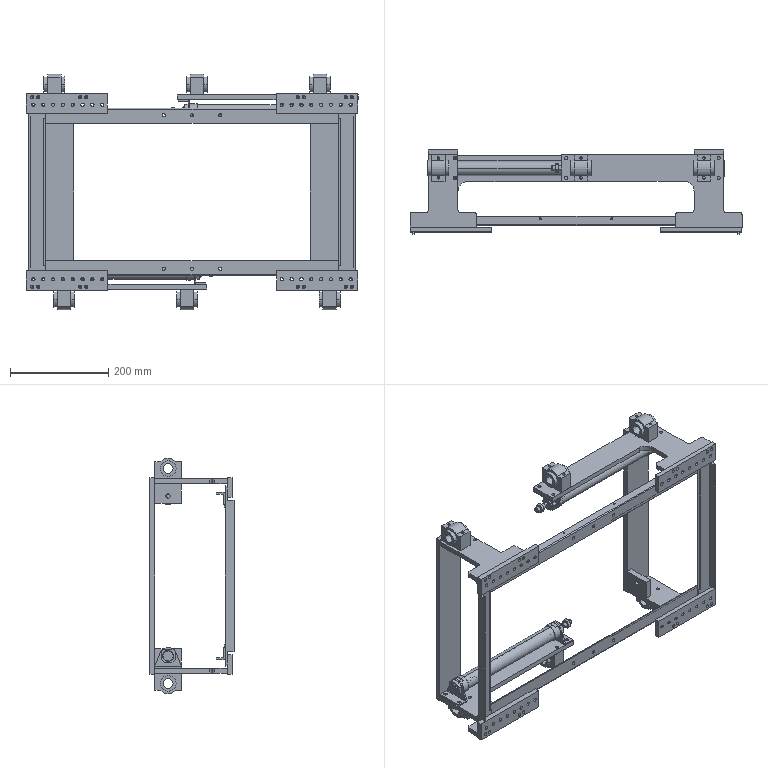Assembly | SolidWorks | mm | 30 component files | 36 solids | 1020 faces | box 675 x 171 x 479 mm | volume 2445017 mm3 | cylinder 492 | plane 356 | cone 140 | torus 32 | commonest cylinder face diameters 6.6 x192 5 x80 32 x32 10 x28 5.2 x24 22 x16 3.3 x16 34 x12
Bill of materials:
AluminumAlloyMiniCylinder-MAL-25x210-S-CM-AIRTAC | 2 | Q235A | Long, slender body of revolution: a plain cylindrical barrel with a wider collar at each end, a short smaller-diameter boss on the rear end, and on the front end a stepped nose with a hex-shaped nut, then a thin protruding rod that carries a second small hex nut and ends in a short stub.
BoxShortLinearBearing-SC20VUU-WERB | 6 |  | Rectangular block with a flat top and a half-round lower side. A cylindrical hub sticks out a short distance from both opposite faces, and a large through-bore runs through the block along the hub axis. Two small holes go down through the top face, one near each end.
CTM-HVS-42-02-27 | 4 | Q235A Cold Rolled Sheet 3mm | L-shaped bent plate bracket. The upright leg tapers to a rounded top and has one large circular hole. The flat base leg is rectangular with two smaller holes. The bend has an inside radius, and the base corners are slightly chamfered.
CTM-HVS-42-02-28 | 2 | Q235A | Thin ring with a large central round bore. The outer profile is a hexagon with its corners cut off by a circle (corner chamfers or rounding), similar in form to a thin jam nut.
CTM-HVS-42-02-29 | 2 | Q235A | Flat plate of uniform thickness with an inverted-L / T-like outline: a long rectangular arm plus a wider foot section at one end. The inside corner is filleted. Four through-holes sit in the face at each end of the long arm, and pairs of holes are drilled into the edge of the foot.
CTM-HVS-42-02-30 | 2 | Q235A | Long, thin rectangular flat plate with five small through-holes near the ends: two at one end plus a third slightly inboard, and two at the opposite end.
CTM-HVS-42-02-31 | 4 | Bakelite | Rectangular flat bar of moderate thickness with a row of eight evenly spaced through-holes along its length. Two extra pairs of holes sit in a second row below.
CTM-HVS-52-OA-02-08-01 | 2 | Q235A | Flat T-shaped plate of uniform thickness. A rectangular stem joins a wider crossbar, with filleted inside corners and rounded outer corners on the crossbar. Four through-holes sit in a rectangular pattern on the stem, and two pairs of holes are drilled into the crossbar's long edge.
CTM-HVS-52-OA-02-14 | 2 | 316L | Long straight member with an L-shaped cross-section: a thin flange plus a perpendicular leg. The leg stops short of both ends, leaving flat end tabs. Each end tab has three small holes in a row.
CTM-HVS-52-OA-02-15 | 2 | 316L | Long straight angle profile. The end view shows an L section with a rounded outer corner, a filleted inner corner, and a step that makes the upright leg thicker below a certain height. Small holes are spaced along the middle of the length on both legs.
CTM-HVS-52-OA-02-16-01 | 2 | Q235A | Solid rectangular block or thick plate with one round through-hole through its large face. The hole sits on the vertical centerline, above center.
Mates:
1. coincident | CTM-HVS-42-02-30-1 face at (-262.307, 82.443, -7.5) dir (0, -1, 0) | CTM-HVS-42-02-29-1 face at (-322.307, 82.443, 5) dir (0, 1, 0)
2. concentric | CTM-HVS-42-02-30-1 face at (-304.807, 92.443, 0) dir (0, 1, 0) r 3.3 | CTM-HVS-42-02-29-1 face at (-304.807, 82.443, 0) dir (0, 1, 0) r 2.5
3. concentric | CTM-HVS-42-02-30-1 face at (-269.807, 92.443, 0) dir (0, 1, 0) r 3.3 | CTM-HVS-42-02-29-1 face at (-269.807, 82.443, 0) dir (0, 1, 0) r 2.5
4. concentric | CTM-HVS-42-02-29-1 face at (-2.307, 75.443, 5) dir (0, 0, 1) r 3.3 | CTM-HVS-42-02-27-1 face at (-2.307, 75.443, 8) dir (0, 0, 1) r 3.3
5. coincident | CTM-HVS-42-02-29-1 face at (-224.807, -64.557, 5) dir (0, 0, 1) | CTM-HVS-42-02-27-1 face at (-14.107, 28.443, 5) dir (0, 0, -1)
6. coincident | AluminumAlloyMiniCylinder-MAL-25x210-S-CM-AIRTAC-1 face at (-17.307, 55.443, 30) dir (1, 0, 0) | CTM-HVS-42-02-27-1 face at (-17.307, 28.443, 47) dir (-1, 0, 0)
7. concentric | AluminumAlloyMiniCylinder-MAL-25x210-S-CM-AIRTAC-1 face at (-272.307, 55.443, 30) dir (1, 0, 0) r 5 | CTM-HVS-42-02-27-1 face at (-20.307, 55.443, 30) dir (1, 0, 0) r 11.5
8. concentric | AluminumAlloyMiniCylinder-MAL-25x210-S-CM-AIRTAC-1 face at (-311.307, 55.443, 30) dir (1, 0, 0) r 11 | CTM-HVS-42-02-27-2 face at (-294.307, 55.443, 30) dir (-1, 0, 0) r 11.5
9. coincident | AluminumAlloyMiniCylinder-MAL-25x210-S-CM-AIRTAC-1 face at (-297.307, 71.605, 31.114) dir (-1, 0, 0) | CTM-HVS-42-02-27-2 face at (-297.307, 82.443, 47) dir (1, 0, 0)
10. coincident | CTM-HVS-42-02-27-1 face at (-14.107, 28.443, 5) dir (0, 0, -1) | CTM-HVS-42-02-27-2 face at (-300.507, 82.443, 5) dir (0, 0, -1)
11. concentric | AluminumAlloyMiniCylinder-MAL-25x210-S-CM-AIRTAC-1 face at (-311.307, 55.443, 30) dir (1, 0, 0) r 11 | CTM-HVS-42-02-28-1 face at (-300.307, 55.443, 30) dir (1, 0, 0) r 11
12. coincident | CTM-HVS-42-02-27-2 face at (-300.307, 82.443, 9.5) dir (-1, 0, 0) | CTM-HVS-42-02-28-1 face at (-300.307, 55.443, 30) dir (1, 0, 0)
13. coincident | CTM-HVS-42-02-29-1 face at (-359.807, -64.557, 5) dir (0, -1, 0) | CTM-HVS-42-02-31-1 face at (-174.807, -64.557, 32.5) dir (0, 1, 0)
14. concentric | CTM-HVS-42-02-29-1 face at (-334.807, -64.557, 0) dir (0, -1, 0) r 2.5 | CTM-HVS-42-02-31-1 face at (-334.807, -74.558, 0) dir (0, 1, 0) r 3.3
15. concentric | CTM-HVS-42-02-29-1 face at (-249.807, -64.557, 0) dir (0, -1, 0) r 2.5 | CTM-HVS-42-02-31-1 face at (-249.807, -74.558, 0) dir (0, 1, 0) r 3.3
16. coincident | CTM-HVS-42-02-29-1 face at (-224.807, -64.557, -5) dir (0, 0, -1) | BoxShortLinearBearing-SC20VUU-WERB-1 face at (-296.007, 82.443, -5) dir (0, 0, 1)
17. concentric | CTM-HVS-42-02-29-1 face at (-282.307, 75.443, -5) dir (0, 0, 1) r 3.3 | BoxShortLinearBearing-SC20VUU-WERB-1 face at (-282.307, 75.443, -47) dir (0, 0, 1) r 2.6
18. concentric | BoxShortLinearBearing-SC20VUU-WERB-2 face at (-32.307, 75.443, -47) dir (0, 0, 1) r 2.6 | CTM-HVS-42-02-29-1 face at (-32.307, 75.443, -5) dir (0, 0, 1) r 3.3
19. coincident | BoxShortLinearBearing-SC20VUU-WERB-2 face at (-46.007, 82.443, -5) dir (0, 0, 1) | BoxShortLinearBearing-SC20VUU-WERB-1 face at (-296.007, 82.443, -5) dir (0, 0, 1)
20. coincident | BoxShortLinearBearing-SC20VUU-WERB-3 face at (243.993, 82.443, -5) dir (0, 0, 1) | CTM-HVS-52-OA-02-08-01-1 face at (277.693, 82.443, -5) dir (0, 0, -1)
21. concentric | BoxShortLinearBearing-SC20VUU-WERB-3 face at (257.693, 75.443, -47) dir (0, 0, 1) r 2.6 | CTM-HVS-52-OA-02-08-01-1 face at (257.693, 75.443, 5) dir (0, 0, 1) r 3.3
22. concentric | BoxShortLinearBearing-SC20VUU-WERB-3 face at (257.693, 35.443, -47) dir (0, 0, 1) r 2.6 | CTM-HVS-52-OA-02-08-01-1 face at (257.693, 35.443, 5) dir (0, 0, 1) r 3.3
23. coincident | CTM-HVS-42-02-29-1 face at (-322.307, -34.557, 5) dir (-1, 0, 0) | CTM-HVS-52-OA-02-08-01-2 face at (-322.307, -34.557, 380) dir (-1, 0, 0)
24. coincident | CTM-HVS-52-OA-02-08-01-2 face at (-359.807, -64.557, 380) dir (0, -1, 0) | CTM-HVS-42-02-31-2 face at (-174.807, -64.557, 352.5) dir (0, 1, 0)
25. concentric | CTM-HVS-52-OA-02-08-01-2 face at (-249.807, -64.557, 385) dir (0, -1, 0) r 2.5 | CTM-HVS-42-02-31-2 face at (-249.807, -64.556, 385) dir (0, -1, 0) r 3.3
26. concentric | CTM-HVS-42-02-31-2 face at (-334.807, -64.556, 385) dir (0, -1, 0) r 3.3 | CTM-HVS-52-OA-02-08-01-2 face at (-334.807, -64.557, 385) dir (0, -1, 0) r 2.5
27. coincident | CTM-HVS-42-02-31-3 face at (130.193, -64.557, 352.5) dir (0, 1, 0) | CTM-HVS-52-OA-02-14-1 face at (310.193, -64.557, 375.5) dir (0, -1, 0)
28. concentric | CTM-HVS-52-OA-02-14-1 face at (300.193, -64.557, 370) dir (0, -1, 0) r 2.5 | CTM-HVS-42-02-31-3 face at (300.193, -64.557, 370) dir (0, 1, 0) r 3.3
29. coincident | CTM-HVS-42-02-30-2 face at (217.693, 82.443, 392.5) dir (0, -1, 0) | CTM-HVS-52-OA-02-08-01-1 face at (217.693, 82.443, 5) dir (0, 1, 0)
30. coincident | CTM-HVS-52-OA-02-08-01-1 face at (277.693, 82.443, 5) dir (0, 0, 1) | CTM-HVS-52-OA-02-16-01-1 face at (217.693, 82.443, 5) dir (0, 0, -1)
31. concentric | CTM-HVS-52-OA-02-08-01-1 face at (223.693, 75.443, 5) dir (0, 0, 1) r 3.3 | CTM-HVS-52-OA-02-16-01-1 face at (223.693, 75.443, 5) dir (0, 0, -1) r 2.5
32. concentric | CTM-HVS-52-OA-02-08-01-1 face at (223.693, 35.443, 5) dir (0, 0, 1) r 3.3 | CTM-HVS-52-OA-02-16-01-1 face at (223.693, 35.443, 5) dir (0, 0, -1) r 2.5
33. coincident | CTM-HVS-42-02-31-1 face at (-174.807, -64.557, 32.5) dir (0, 1, 0) | CTM-HVS-52-OA-02-14-2 face at (-354.807, -64.557, 9.5) dir (0, -1, 0)
34. concentric | CTM-HVS-52-OA-02-14-2 face at (-344.807, -64.557, 370) dir (0, -1, 0) r 2.5 | CTM-HVS-42-02-31-2 face at (-344.807, -74.557, 370) dir (0, -1, 0) r 3.3
35. distance | CTM-HVS-52-OA-02-15-2 face at (297.693, -56.557, 332.5) dir (0, 0, -1) | CTM-HVS-52-OA-02-15-1 face at (-342.307, -56.557, 52.5) dir (0, 0, 1)
36. concentric | CTM-HVS-52-OA-02-08-01-1 face at (232.693, 82.443, 0) dir (0, 1, 0) r 2.5 | CTM-HVS-42-02-30-2 face at (232.693, 82.443, 0) dir (0, 1, 0) r 3.3
37. concentric | BoxShortLinearBearing-SC20VUU-WERB-2 face at (-53.307, 55.443, -26) dir (1, 0, 0) r 10 | BoxShortLinearBearing-SC20VUU-WERB-3 face at (236.693, 55.443, -26) dir (1, 0, 0) r 10
38. concentric | CTM-HVS-52-OA-02-08-01-1 face at (267.693, 82.443, 0) dir (0, 1, 0) r 2.5 | CTM-HVS-42-02-30-2 face at (267.693, 82.443, 0) dir (0, 1, 0) r 3.3
39. coincident | CTM-HVS-52-OA-02-08-01-1 face at (315.193, -64.557, 5) dir (0, -1, 0) | CTM-HVS-42-02-31-4 face at (130.193, -64.557, 32.5) dir (0, 1, 0)
40. concentric | CTM-HVS-52-OA-02-14-1 face at (300.193, -64.557, 15) dir (0, -1, 0) r 2.5 | CTM-HVS-42-02-31-4 face at (300.193, -74.557, 15) dir (0, -1, 0) r 3.3
41. concentric | CTM-HVS-52-OA-02-14-1 face at (280.193, -64.557, 15) dir (0, -1, 0) r 2.5 | CTM-HVS-42-02-31-4 face at (280.193, -74.557, 15) dir (0, -1, 0) r 3.3
42. coincident | CTM-HVS-42-02-31-1 face at (-174.807, -74.557, 32.5) dir (0, -1, 0) | CTM-HVS-42-02-31-4 face at (130.193, -74.557, 32.5) dir (0, -1, 0)
43. coincident | CTM-HVS-42-02-30-2 face at (217.693, 82.443, 392.5) dir (0, -1, 0) | CTM-HVS-42-02-29-2 face at (277.693, 82.443, 380) dir (0, 1, 0)
44. concentric | CTM-HVS-42-02-30-2 face at (260.193, 92.443, 385) dir (0, 1, 0) r 3.3 | CTM-HVS-42-02-29-2 face at (260.193, 82.443, 385) dir (0, 1, 0) r 2.5
45. concentric | CTM-HVS-42-02-30-2 face at (225.193, 92.443, 385) dir (0, 1, 0) r 3.3 | CTM-HVS-42-02-29-2 face at (225.193, 82.443, 385) dir (0, 1, 0) r 2.5
46. concentric | CTM-HVS-42-02-31-1 face at (-324.807, -64.557, 15) dir (0, 1, 0) r 3.3 | CTM-HVS-52-OA-02-14-2 face at (-324.807, -64.557, 15) dir (0, -1, 0) r 2.5
47. coincident | CTM-HVS-42-02-30-1 face at (-262.307, 82.443, -7.5) dir (0, -1, 0) | CTM-HVS-52-OA-02-08-01-2 face at (-262.307, 82.443, 380) dir (0, 1, 0)
48. coincident | CTM-HVS-52-OA-02-15-1 face at (297.693, -60.557, 52.5) dir (0, -1, 0) | CTM-HVS-52-OA-02-14-1 face at (310.193, -60.557, 375.5) dir (0, 1, 0)
49. coincident | CTM-HVS-52-OA-02-14-1 face at (310.193, -64.557, 375.5) dir (0, -1, 0) | CTM-HVS-42-02-31-4 face at (130.193, -64.557, 32.5) dir (0, 1, 0)
50. width | CTM-HVS-42-02-29-1 face at (-224.807, -64.557, -5) dir (0, 0, -1) | CTM-HVS-52-OA-02-08-01-2 face at (-322.307, 82.443, 390) dir (0, 0, 1) | CTM-HVS-52-OA-02-15-2 face at (297.693, -56.557, 362.5) dir (0, 0, 1) | CTM-HVS-52-OA-02-15-1 face at (-342.307, -56.557, 22.5) dir (0, 0, -1)
51. width | CTM-HVS-52-OA-02-14-1 face at (310.193, -64.557, 9.5) dir (1, 0, 0) | CTM-HVS-52-OA-02-14-2 face at (-354.807, -64.557, 375.5) dir (-1, 0, 0) | CTM-HVS-52-OA-02-15-2 face at (-342.307, -56.557, 362.5) dir (-1, 0, 0) | CTM-HVS-52-OA-02-15-2 face at (297.693, -56.557, 362.5) dir (1, 0, 0)
52. coincident | CTM-HVS-52-OA-02-08-01-2 face at (-322.307, 82.443, 390) dir (0, 0, 1) | BoxShortLinearBearing-SC20VUU-WERB-4 face at (-288.607, 82.443, 390) dir (0, 0, -1)
53. concentric | CTM-HVS-52-OA-02-08-01-2 face at (-302.307, 75.443, 380) dir (0, 0, -1) r 3.3 | BoxShortLinearBearing-SC20VUU-WERB-4 face at (-302.307, 75.443, 432) dir (0, 0, -1) r 2.6
54. concentric | CTM-HVS-52-OA-02-08-01-2 face at (-302.307, 35.443, 380) dir (0, 0, -1) r 3.3 | BoxShortLinearBearing-SC20VUU-WERB-4 face at (-302.307, 35.443, 432) dir (0, 0, -1) r 2.6
55. coincident | CTM-HVS-42-02-29-2 face at (180.193, -64.557, 390) dir (0, 0, 1) | BoxShortLinearBearing-SC20VUU-WERB-6 face at (1.393, 82.443, 390) dir (0, 0, -1)
56. concentric | CTM-HVS-42-02-29-2 face at (-12.307, 75.443, 390) dir (0, 0, -1) r 3.3 | BoxShortLinearBearing-SC20VUU-WERB-6 face at (-12.307, 75.443, 432) dir (0, 0, -1) r 2.6
57. concentric | CTM-HVS-42-02-29-2 face at (-12.307, 35.443, 390) dir (0, 0, -1) r 3.3 | BoxShortLinearBearing-SC20VUU-WERB-6 face at (-12.307, 35.443, 432) dir (0, 0, -1) r 2.6
58. coincident | CTM-HVS-52-OA-02-08-01-2 face at (-322.307, 82.443, 380) dir (0, 0, -1) | CTM-HVS-52-OA-02-16-01-2 face at (-262.307, 82.443, 380) dir (0, 0, 1)
59. coincident | CTM-HVS-52-OA-02-08-01-2 face at (-262.307, -34.557, 380) dir (1, 0, 0) | CTM-HVS-52-OA-02-16-01-2 face at (-262.307, 28.443, 340) dir (1, 0, 0)
60. concentric | CTM-HVS-52-OA-02-08-01-2 face at (-268.307, 75.443, 380) dir (0, 0, -1) r 3.3 | CTM-HVS-52-OA-02-16-01-2 face at (-268.307, 75.443, 380) dir (0, 0, 1) r 2.5
61. coincident | CTM-HVS-42-02-29-2 face at (180.193, -64.557, 380) dir (0, 0, -1) | CTM-HVS-42-02-27-3 face at (-30.507, 28.443, 380) dir (0, 0, 1)
62. concentric | CTM-HVS-42-02-29-2 face at (-42.307, 75.443, 380) dir (0, 0, -1) r 3.3 | CTM-HVS-42-02-27-3 face at (-42.307, 75.443, 377) dir (0, 0, -1) r 3.3
63. concentric | CTM-HVS-42-02-29-2 face at (-42.307, 35.443, 380) dir (0, 0, -1) r 3.3 | CTM-HVS-42-02-27-3 face at (-42.307, 35.443, 377) dir (0, 0, -1) r 3.3
64. concentric | CTM-HVS-42-02-27-3 face at (-24.307, 55.443, 355) dir (-1, 0, 0) r 11.5 | AluminumAlloyMiniCylinder-MAL-25x210-S-CM-AIRTAC-2 face at (227.693, 55.443, 355) dir (-1, 0, 0) r 5
65. coincident | CTM-HVS-42-02-27-3 face at (-27.307, 28.443, 338) dir (1, 0, 0) | AluminumAlloyMiniCylinder-MAL-25x210-S-CM-AIRTAC-2 face at (-27.307, 55.443, 355) dir (-1, 0, 0)
66. coincident | CTM-HVS-42-02-29-2 face at (180.193, -64.557, 380) dir (0, 0, -1) | CTM-HVS-42-02-27-4 face at (255.893, 82.443, 380) dir (0, 0, 1)
67. coincident | CTM-HVS-42-02-29-2 edge at (267.693, 75.443, 380) dir (0, 0, -1) r 3.3 | CTM-HVS-42-02-27-4 face at (267.693, 75.443, 377) dir (0, 0, -1) r 3.3
68. concentric | CTM-HVS-42-02-29-2 face at (267.693, 35.443, 380) dir (0, 0, -1) r 3.3 | CTM-HVS-42-02-27-4 face at (267.693, 35.443, 377) dir (0, 0, -1) r 3.3
69. concentric | AluminumAlloyMiniCylinder-MAL-25x210-S-CM-AIRTAC-2 face at (266.693, 55.443, 355) dir (-1, 0, 0) r 11 | CTM-HVS-42-02-28-2 face at (262.693, 55.443, 355) dir (1, 0, 0) r 11
70. coincident | CTM-HVS-42-02-27-4 face at (255.693, 82.443, 375.5) dir (1, 0, 0) | CTM-HVS-42-02-28-2 face at (255.693, 55.443, 355) dir (-1, 0, 0)
71. distance | CTM-HVS-52-OA-02-08-01-1 face at (217.693, -34.557, 5) dir (-1, 0, 0) | CTM-HVS-42-02-29-1 face at (7.693, 82.443, 5) dir (1, 0, 0)
72. concentric | CTM-HVS-42-02-31-3 face at (302.693, -74.558, 385) dir (0, 1, 0) r 3.3 | CTM-HVS-42-02-29-2 face at (302.693, -64.557, 385) dir (0, -1, 0) r 2.5
73. concentric | CTM-HVS-42-02-31-3 face at (290.193, -74.558, 385) dir (0, 1, 0) r 3.3 | CTM-HVS-42-02-29-2 face at (290.193, -64.557, 385) dir (0, -1, 0) r 2.5